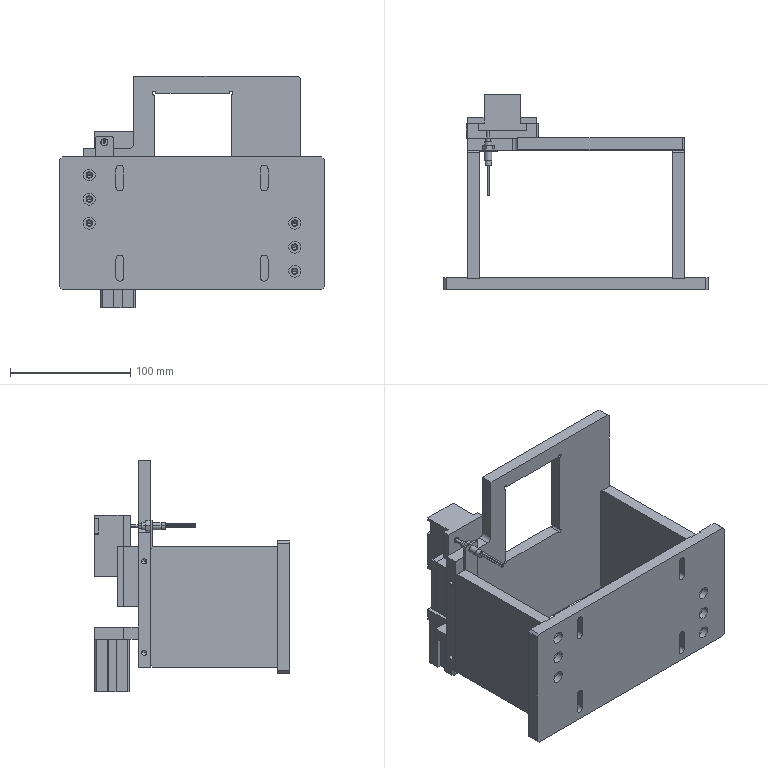Assembly | SolidWorks | mm | 13 component files | 13 solids | 443 faces | box 220 x 162.5 x 192.28 mm | volume 798852 mm3 | cylinder 188 | plane 179 | cone 66 | torus 10 | commonest cylinder face diameters 4.2 x36 0.4 x18 10 x12 5.3 x12 5.5 x10 6 x10 6.6 x8 1 x8
Bill of materials:
610FiberOptic | 1 |  | Axially stepped cylindrical body with a hexagonal flange near one end, a smaller cylindrical spigot on the hex side, and two thin parallel rods coming out of the opposite end.
AirCylinderSupportBlock2 | 1 | 1023 Carbon Steel Plate (SS) | Inverted-T shaped prismatic block. It has a large through bore and two small holes on the main face, plus two holes through the long base bar running crosswise to the bore.
BottomSupport | 1 |  | Thin rectangular plate with chamfered corners. It has four elongated slots and two groups of three small round holes near opposite ends.
GuideRailPlane | 1 |  | Flat plate with an L-shaped (notched-corner) outline and a rectangular window cutout with small corner relief holes. There are small holes in one edge face.
SidePlate | 2 |  | Thick rectangular plate with one chamfered corner edge. It has three small holes in a row on one narrow edge face.
FiberOpticBracket | 1 |  | Thin flat rectangular tab with fully rounded corners and a single round through hole near one end.
PusherBlockSlideSeat | 1 |  | Rectangular block with a wide shallow channel across one face, giving a U-shaped cross section. Eight through holes form a symmetric pattern on the main face.
PusherBlockSlideSeatCoverPlate | 1 |  | Rectangular bar/spacer block with two round through holes near its ends, offset slightly from the width centerline.
PusherBlockSlideSeatCoverPlate3 | 1 |  | Rectangular bar/spacer block with two round through holes near its ends, offset slightly from the width centerline.
PusherSeat | 1 | 201 Annealed Stainless Steel (SS) | Rectangular block with a step or flange along its base, giving an inverted-T profile in one view. There is a single small hole near one top corner of one face.
SDA_16x2525_b | 1 |  | Square prismatic extruded body with chamfered corners and longitudinal slots on its sides. One end face has a central protruding round boss with a hole, an annular groove, and two counterbored through holes at opposite corners.
SDA_16x2525_r | 1 |  | Long cylindrical shaft with a flat at one end and a small axial hole in that end. The other end has a larger disc-like head with two radial flanges separated by a groove.
Mates:
1. coincident | PusherBlockSlideSeat-1 face at (-26.915, 5.195, 122.481) dir (0, 1, 0) | PusherSeat-1 face at (8.085, 5.195, 76.579) dir (0, -1, 0)
2. coincident | PusherBlockSlideSeat-1 face at (13.085, 5.195, 44.293) dir (-1, 0, 0) | PusherSeat-1 face at (13.085, 5.195, 123.189) dir (1, 0, 0)
3. coincident | PusherBlockSlideSeat-1 face at (-35.915, 11.195, 101.579) dir (0, 1, 0) | PusherBlockSlideSeatCoverPlate-1 face at (-21.915, 11.195, 101.579) dir (0, -1, 0)
4. coincident | PusherBlockSlideSeat-1 face at (-35.915, 11.195, 51.579) dir (-1, 0, 0) | PusherBlockSlideSeatCoverPlate-1 face at (-35.915, 16.195, 101.579) dir (-1, 0, 0)
5. coincident | PusherBlockSlideSeat-1 face at (-35.915, 11.195, 51.579) dir (0, 0, -1) | PusherBlockSlideSeatCoverPlate-1 face at (-35.915, 16.195, 51.579) dir (0, 0, -1)
6. coincident | PusherBlockSlideSeat-1 face at (22.085, 11.195, 51.579) dir (1, 0, 0) | PusherBlockSlideSeatCoverPlate3-1 face at (22.085, 16.195, 51.579) dir (1, 0, 0)
7. coincident | PusherBlockSlideSeat-1 face at (-35.915, 11.195, 51.579) dir (0, 0, -1) | PusherBlockSlideSeatCoverPlate3-1 face at (22.085, 16.195, 51.579) dir (0, 0, -1)
8. coincident | PusherBlockSlideSeat-1 face at (-35.915, 11.195, 101.579) dir (0, 1, 0) | PusherBlockSlideSeatCoverPlate3-1 face at (8.085, 11.195, 51.579) dir (0, -1, 0)
9. distance | PusherSeat-1 face at (-21.915, 35.195, 76.579) dir (0, 0, -1) | PusherBlockSlideSeat-1 face at (-35.915, 11.195, 51.579) dir (0, 0, -1)
10. coincident | PusherBlockSlideSeat-1 face at (-35.915, -1.305, 101.579) dir (0, -1, 0) | AssemblyCylinderBracket54-1/GuideRailPlane-1 face at (54.585, -1.305, 87.359) dir (0, 1, 0)
11. distance | PusherBlockSlideSeat-1 face at (-35.915, 11.195, 51.579) dir (0, 0, -1) | AssemblyCylinderBracket54-1/GuideRailPlane-1 face at (145.085, -1.305, 1.359) dir (0, 0, -1)
12. concentric | PusherSeat-1 face at (-6.915, 20.195, 76.579) dir (0, 0, -1) r 1.25 | AirCylinderSupportBlock2-1 face at (-6.915, 20.195, 24.579) dir (0, 0, 1) r 6.5
13. coincident | AssemblyCylinderBracket54-1/GuideRailPlane-1 face at (54.585, -1.305, 87.359) dir (0, 1, 0) | AirCylinderSupportBlock2-1 face at (-36.915, -1.305, 24.579) dir (0, -1, 0)
14. distance | AirCylinderSupportBlock2-1 face at (-21.915, 35.195, 34.579) dir (0, 0, 1) | PusherBlockSlideSeat-1 face at (-35.915, 11.195, 51.579) dir (0, 0, -1)
15. concentric | AirCylinderSupportBlock2-1 face at (-16.815, 30.095, 24.579) dir (0, 0, -1) r 1.65 | SDA_16x25_0-1/SDA_16x2525_b-1 face at (-16.815, 30.095, 2.829) dir (0, 0, 1) r 3.25
16. parallel | AirCylinderSupportBlock2-1 face at (2.985, 10.295, 24.579) dir (0, 0, -1) r 1.65 | SDA_16x25_0-1/SDA_16x2525_b-1 face at (2.984, 10.296, 2.829) dir (0, 0, 1) r 3.25
17. coincident | AirCylinderSupportBlock2-1 face at (-21.915, 35.195, 24.579) dir (0, 0, -1) | SDA_16x25_0-1/SDA_16x2525_b-1 face at (7.384, 23.995, 24.579) dir (0, 0, 1)
18. coincident | AssemblyCylinderBracket54-1/GuideRailPlane-1 face at (54.585, -11.305, 87.359) dir (0, -1, 0) | FiberOpticBracket-1 face at (-25.865, -11.305, 83.579) dir (0, 1, 0)
19. concentric | FiberOpticBracket-1 face at (-18.365, -21.305, 118.579) dir (0, 1, 0) r 3 | 610FiberOptic-1 face at (-18.365, -24.305, 118.579) dir (0, 1, 0) r 3
20. coincident | FiberOpticBracket-1 face at (-25.865, -11.305, 83.579) dir (0, 1, 0) | 610FiberOptic-1 face at (-18.365, -11.305, 118.579) dir (0, -1, 0)
21. parallel | AirCylinderSupportBlock2-1 face at (8.085, 35.195, 24.579) dir (0, 1, 0) | SDA_16x25_0-1/SDA_16x2525_b-1 face at (-19.916, 34.695, -18.921) dir (0, 1, 0)
22. coincident | PusherBlockSlideSeat-1 face at (-35.915, 11.195, 51.579) dir (-1, 0, 0) | AssemblyCylinderBracket54-1/GuideRailPlane-1 face at (-35.915, -1.305, 1.359) dir (-1, 0, 0)
23. distance | FiberOpticBracket-1 face at (-25.865, -11.305, 83.579) dir (-1, 0, 0) | AssemblyCylinderBracket54-1/GuideRailPlane-1 face at (-35.915, -1.305, 1.359) dir (-1, 0, 0)
24. distance | FiberOpticBracket-1 face at (-25.865, -11.305, 123.579) dir (0, 0, 1) | AssemblyCylinderBracket54-1/GuideRailPlane-1 face at (-35.915, -11.305, 113.359) dir (0, 0, 1)
25. width | SidePlate-1 face at (-73.629, -55.833, 251) dir (0, -1, 0) | SidePlate-1 face at (-73.629, 44.167, 251) dir (0, 1, 0) | BottomSupport-1 face at (-93.129, 49.167, 145) dir (0, 1, 0) | BottomSupport-1 face at (-93.129, -60.833, 145) dir (0, -1, 0)
26. width | SidePlate-2 face at (107.371, -55.833, 251) dir (0, -1, 0) | SidePlate-2 face at (107.371, 44.167, 251) dir (0, 1, 0) | BottomSupport-1 face at (-93.129, 49.167, 145) dir (0, 1, 0) | BottomSupport-1 face at (-93.129, -60.833, 145) dir (0, -1, 0)
27. coincident | SidePlate-2 face at (107.371, 44.167, 251) dir (0, 1, 0) | GuideRailPlane-1 face at (107.371, 44.167, 261) dir (0, 1, 0)
28. coincident | GuideRailPlane-1 face at (16.871, -41.833, 251) dir (0, 0, -1) | AssemblyCylinderBracket54 face at (-4.129, 10.167, 429.58) dir (0, 0, 1)
29. width | AssemblyCylinderBracket54 face at (-4.129, 10.167, 424.58) dir (-1, 0, 0) | AssemblyCylinderBracket54 face at (37.871, 10.167, 424.58) dir (1, 0, 0) | GuideRailPlane-1 face at (-73.629, 44.167, 261) dir (-1, 0, 0) | GuideRailPlane-1 face at (107.371, 44.167, 261) dir (1, 0, 0)
30. distance | SidePlate-1 face at (-73.629, -55.833, 251) dir (0, -1, 0) | AssemblyCylinderBracket54 face at (-4.129, 5.167, 396.58) dir (0, -1, 0)
31. coincident | GuideRailPlane-1 face at (16.871, -41.833, 251) dir (0, 0, -1) | AssemblyCylinderBracket54 face at (-8.634, -32.833, 429.58) dir (0, 0, 1)
32. coincident | GuideRailPlane-1 face at (107.371, -127.833, 261) dir (0, -1, 0) | AssemblyCylinderBracket54 face at (-9.129, -105.833, 424.33) dir (0, -1, 0)
33. distance | AssemblyCylinderBracket54 face at (-9.129, -32.833, 425.58) dir (-1, 0, 0) | GuideRailPlane-1 face at (-73.629, 44.167, 261) dir (-1, 0, 0)
34. coincident | GuideRailPlane-1 face at (16.871, -41.833, 251) dir (0, 0, -1) | AssemblyCylinderBracket54 face at (31.366, -32.833, 429.58) dir (0, 0, 1)
35. coincident | GuideRailPlane-1 face at (107.371, -127.833, 261) dir (0, -1, 0) | AssemblyCylinderBracket54 face at (30.871, -105.833, 424.33) dir (0, -1, 0)
36. distance | AssemblyCylinderBracket54 face at (42.871, -32.833, 429.085) dir (1, 0, 0) | GuideRailPlane-1 face at (107.371, 44.167, 261) dir (1, 0, 0)
37. distance | AssemblyCylinderBracket54 face at (-9.129, -25.833, 430.58) dir (-1, 0, 0) | GuideRailPlane-1 face at (-73.629, 44.167, 261) dir (-1, 0, 0)
38. coincident | GuideRailPlane-1 face at (107.371, -127.833, 261) dir (0, -1, 0) | AssemblyCylinderBracket54 face at (2.871, -105.833, 430.58) dir (0, -1, 0)
39. coincident | GuideRailPlane-1 face at (107.371, -127.833, 261) dir (0, -1, 0) | AssemblyCylinderBracket54 face at (42.871, -105.833, 430.58) dir (0, -1, 0)
40. distance | AssemblyCylinderBracket54 face at (42.871, -25.833, 430.58) dir (1, 0, 0) | GuideRailPlane-1 face at (107.371, 44.167, 261) dir (1, 0, 0)
41. coincident | AssemblyCylinderBracket54 face at (16.871, -97.933, 320.76) dir (0, 0, -1) | AssemblyCylinderBracket54 face at (13.871, -81.933, 320.76) dir (0, 0, 1)
42. width | AssemblyCylinderBracket54 face at (27.971, -81.933, 320.16) dir (1, 0, 0) | AssemblyCylinderBracket54 face at (5.771, -81.933, 305.06) dir (-1, 0, 0) | AssemblyCylinderBracket54 face at (-3.629, -82.133, 325.76) dir (-1, 0, 0) | AssemblyCylinderBracket54 face at (37.371, -97.733, 325.76) dir (1, 0, 0)
43. coincident | AssemblyCylinderBracket54 face at (37.171, -81.933, 325.76) dir (0, 1, 0) | AssemblyCylinderBracket54 face at (23.671, -81.933, 320.56) dir (0, 1, 0)
44. coincident | AssemblyCylinderBracket54 face at (16.871, -142.657, 314.383) dir (0, 1, 0) | AssemblyCylinderBracket54 face at (16.871, -142.657, 312.61) dir (0, -1, 0)
45. coincident | AssemblyCylinderBracket54 face at (21.871, -124.933, 308.96) dir (0, 1, 0) | AssemblyCylinderBracket54 face at (23.671, -124.933, 320.56) dir (0, -1, 0)
46. width | SidePlate-1 face at (-73.629, -5.833, 197.5) dir (-1, 0, 0) | SidePlate-2 face at (107.371, -5.833, 197.5) dir (1, 0, 0) | BottomSupport-1 face at (-93.129, 49.167, 145) dir (-1, 0, 0) | BottomSupport-1 face at (126.871, 49.167, 145) dir (1, 0, 0)
47. coincident | BottomSupport-1 face at (-73.629, 49.167, 144) dir (0, 0, 1) | SidePlate-1 face at (-73.629, -55.833, 144) dir (0, 0, -1)
48. coincident | BottomSupport-1 face at (97.371, 49.167, 144) dir (0, 0, 1) | SidePlate-2 face at (107.371, 44.167, 144) dir (0, 0, -1)
49. coincident | GuideRailPlane-1 face at (42.871, -20.833, 430.58) dir (0, 0, -1) | AssemblyCylinderBracket54 face at (36.871, -65.833, 430.58) dir (0, 0, 1)
50. coincident | GuideRailPlane-1 face at (-9.129, -20.833, 430.58) dir (0, 0, -1) | AssemblyCylinderBracket54 face at (-3.129, -65.833, 430.58) dir (0, 0, 1)
51. coincident | BottomSupport-1 face at (-73.629, 49.167, 145) dir (1, 0, 0) | SidePlate-1 face at (-73.629, -5.833, 197.5) dir (-1, 0, 0)
52. coincident | SidePlate-1 face at (-73.629, -55.833, 251) dir (0, 0, 1) | GuideRailPlane-1 face at (16.871, -41.833, 251) dir (0, 0, -1)
53. coincident | SidePlate-1 face at (-73.629, -5.833, 197.5) dir (-1, 0, 0) | GuideRailPlane-1 face at (-73.629, 44.167, 261) dir (-1, 0, 0)
54. coincident | SDA_16x2525_b-1 axis at (-80.9, 0, 0) dir (1, 0, 0) | SDA_16x2525_r-1 axis at (80.9, 0, 0) dir (-1, 0, 0)
55. angle | SDA_16x2525_r-1 plane at (0, 0, 0) dir (0, 0, -1) | SDA_16x2525_b-1 plane at (0, 0, 0) dir (0, 1, 0)